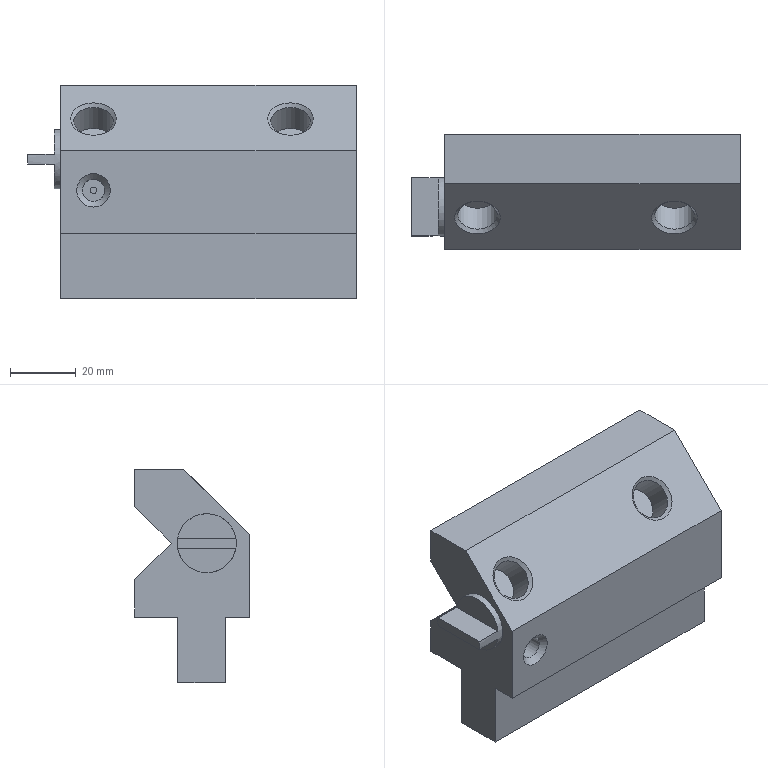Component | NX | MAGNETIC_BASE | 1 solid | 34 faces | volume 135400 mm3 | plane 24 | cylinder 6 | cone 4 | commonest cylinder face diameters 12 x3 18 x1 6.8 x1 2 x1